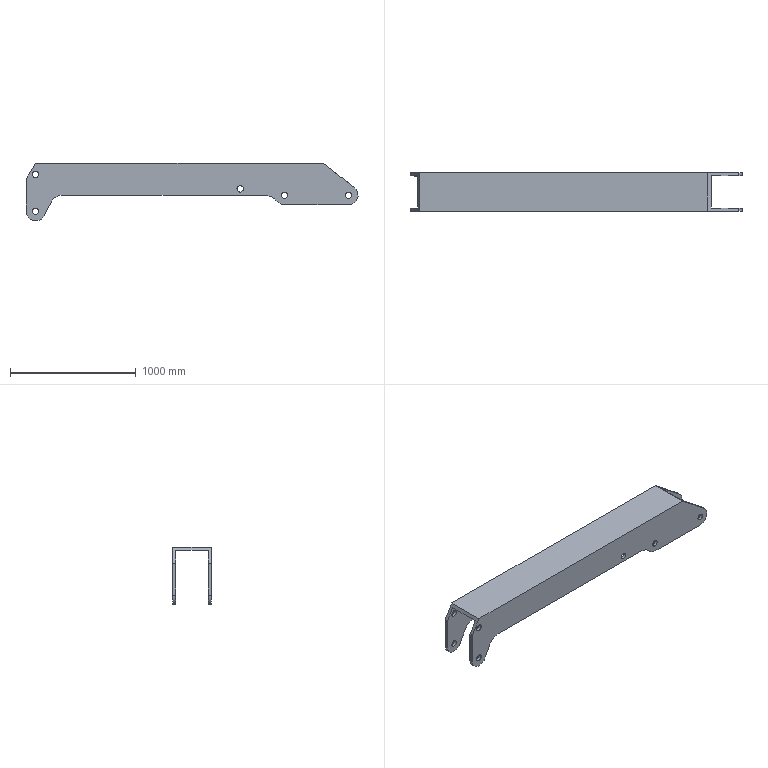Component | NX | EXT_ARM | 1 solid | 36 faces | volume 50397196 mm3 | cylinder 20 | plane 16 | commonest cylinder face diameters 50.8 x10 152.4 x6 262 x2 208 x2